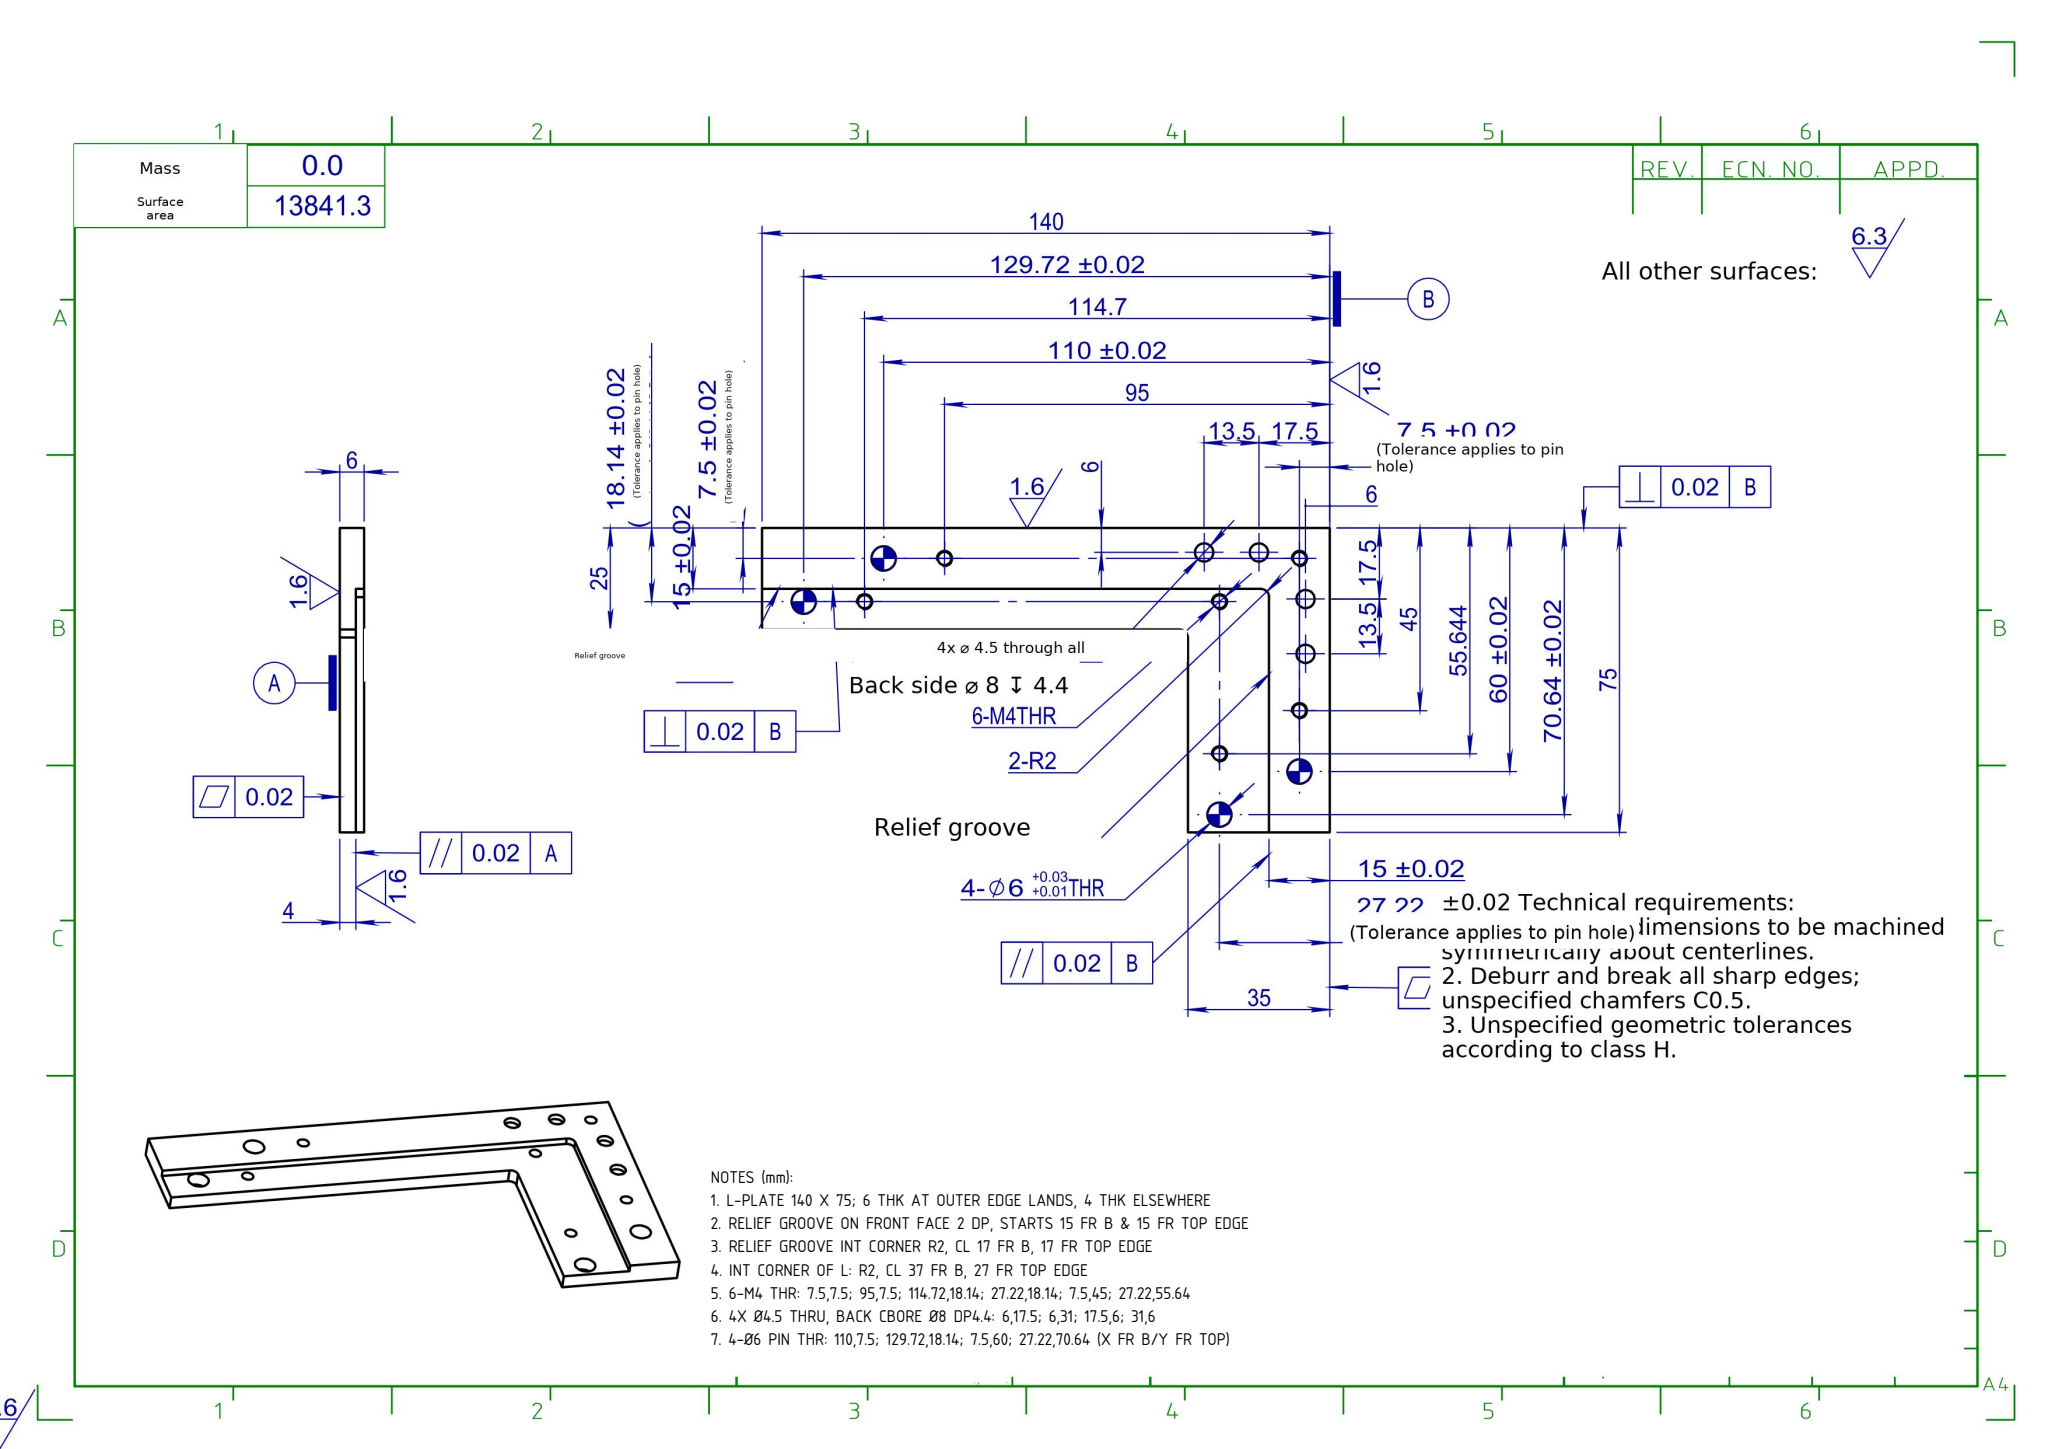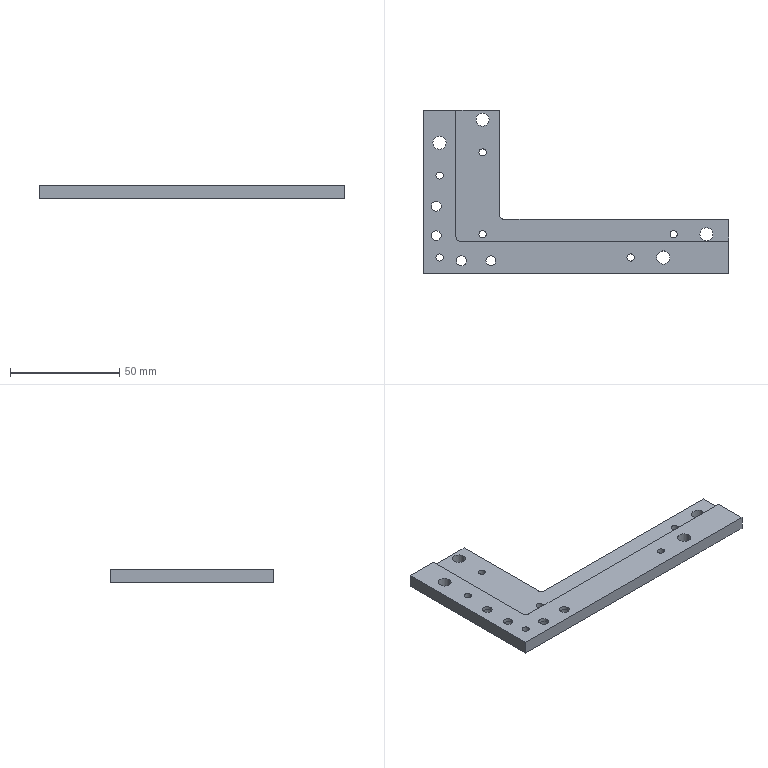Part | SolidWorks | mm | 1 solid | 53 faces | box 140 x 75 x 6 mm | volume 25197 mm3 | cylinder 38 | plane 15 | commonest cylinder face diameters 3.3 x12 6 x8 8 x8 4.5 x8 4 x2
Drawing notes:
L-PLATE 140 X 75; 6 THK AT OUTER EDGE LANDS, 4 THK ELSEWHERE | from the solid: bbox 140x75x6; z planes 0/4/6; x=15 & y=15 planes bound 6 thk land
RELIEF GROOVE ON FRONT FACE 2 DP, STARTS 15 FR B & 15 FR TOP EDGE | from the solid: x=15 & y=15 planes with z=4 face: 6 thk land, 4 thk relieved area = 2 dp
RELIEF GROOVE INT CORNER R2, CL 17 FR B, 17 FR TOP EDGE | from the solid: cyl dia4.0 axis z at (17,17) len 2.0 in 2 dp recess
INT CORNER OF L: R2, CL 37 FR B, 27 FR TOP EDGE | from the solid: cyl dia4.0 axis z at (37,27) len 4.0 tangent to x=35 & y=25 planes
6-M4 THR: 7.5,7.5; 95,7.5; 114.72,18.14; 27.22,18.14; 7.5,45; 27.22,55.64 | from the solid: dia3.3 axis z at listed X(fr B),Y(fr top edge) positions
4X Ø4.5 THRU, BACK CBORE Ø8 DP4.4: 6,17.5; 6,31; 17.5,6; 31,6 | from the solid: dia4.5 len1.6 + dia8.0 len4.4 at (6,17.5),(6,31),(17.5,6),(31,6)
4-Ø6 PIN THR: 110,7.5; 129.72,18.14; 7.5,60; 27.22,70.64 (X FR B/Y FR TOP) | from the solid: dia6.0 axis z at (110,7.5),(129.72,18.14),(7.5,60),(27.22,70.64)
build123d program:
from build123d import *

# Parameters (mm, degrees)
SKETCH1_W                                            = 140
SKETCH1_H                                            = 75
BOSS_EXTRUDE1_DEPTH                                  = 3
SKETCH2_W                                            = 125
SKETCH2_H                                            = 60
CUT_EXTRUDE1_DEPTH                                   = 80.638
BOSS_EXTRUDE2_DEPTH                                  = 8
POST_HOLE_FOR_M4_HEX_SOCKET_HEAD_CAP_SCR_D           = 4.5
POST_HOLE_FOR_M4_HEX_SOCKET_HEAD_CAP_SCR_CBORE_D     = 8
POST_HOLE_FOR_M4_HEX_SOCKET_HEAD_CAP_SCR_CBORE_DEPTH = 4.4
M4_TAPPED_HOLE_3_D                                   = 3.3
SKETCH20_R                                           = 3
CUT_EXTRUDE4_DEPTH                                   = 80.814
CUT_EXTRUDE5_DEPTH                                   = 4
FILLET1_R                                            = 2
FILLET2_R                                            = 2


with BuildPart() as part:
    # Sketch1 → Boss-Extrude1 (new, symmetric)
    with BuildSketch(Plane.XY):
        Rectangle(SKETCH1_W, SKETCH1_H)
    extrude(amount=BOSS_EXTRUDE1_DEPTH, both=True)

    # Sketch2 → Cut-Extrude1 (cut, through all)
    with BuildSketch(Plane.XY.offset(3)):
        with Locations((7.5, 7.5)):
            Rectangle(SKETCH2_W, SKETCH2_H)
    extrude(amount=-CUT_EXTRUDE1_DEPTH, mode=Mode.SUBTRACT)

    # Sketch9 → Boss-Extrude2 (add)
    with BuildSketch(Plane(origin=(0, 0, -3), x_dir=(-1, 0, 0), z_dir=(0, 0, -1))):
        Polygon((-70, -22.5), (55, -22.5), (55, 37.5), (35, 37.5), (35, -12.5), (-70, -12.5), align=None)
    extrude(amount=-BOSS_EXTRUDE2_DEPTH)

    # Post Hole for M4 Hex Socket Head Cap Scr (through all)
    with Locations(Plane(origin=(0, 0, -3), x_dir=(-1, 0, 0), z_dir=(0, 0, -1))):
        with Locations((39, -31.5), (52.5, -31.5), (64, -20), (64, -6.5)):
            CounterBoreHole(POST_HOLE_FOR_M4_HEX_SOCKET_HEAD_CAP_SCR_D / 2, POST_HOLE_FOR_M4_HEX_SOCKET_HEAD_CAP_SCR_CBORE_D / 2, POST_HOLE_FOR_M4_HEX_SOCKET_HEAD_CAP_SCR_CBORE_DEPTH)

    # M4 Tapped Hole 3 (through all)
    with Locations(Plane(origin=(0, 0, -3), x_dir=(-1, 0, 0), z_dir=(0, 0, -1))):
        with Locations((62.5, 7.5), (62.5, -30), (-25, -30), (-44.721, -19.356), (42.779, -19.356), (42.779, 18.144)):
            Hole(M4_TAPPED_HOLE_3_D / 2)

    # Sketch20 → Cut-Extrude4 (cut, through all)
    with BuildSketch(Plane(origin=(0, 0, -3), x_dir=(-1, 0, 0), z_dir=(0, 0, -1))):
        with Locations((-40, -30)):
            Circle(SKETCH20_R)
        with Locations((-59.721, -19.356)):
            Circle(SKETCH20_R)
        with Locations((62.5, 22.5)):
            Circle(SKETCH20_R)
        with Locations((42.779, 33.144)):
            Circle(SKETCH20_R)
    extrude(amount=-CUT_EXTRUDE4_DEPTH, mode=Mode.SUBTRACT)

    # Sketch21 → Cut-Extrude5 (cut)
    with BuildSketch(Plane.XY.offset(5)):
        Polygon((70, -22.5), (70, -12.5), (-35, -12.5), (-35, 37.5), (-55, 37.5), (-55, -22.5), align=None)
    extrude(amount=-CUT_EXTRUDE5_DEPTH, mode=Mode.SUBTRACT)

    # Fillet1
    fillet1_edges = [part.edges().sort_by_distance(p)[0] for p in [
        (-55, -22.5, 2),
    ]]
    fillet(fillet1_edges, radius=FILLET1_R)

    # Fillet2
    fillet2_edges = [part.edges().sort_by_distance(p)[0] for p in [
        (-35, -12.5, -1),
    ]]
    fillet(fillet2_edges, radius=FILLET2_R)


solid = part.part